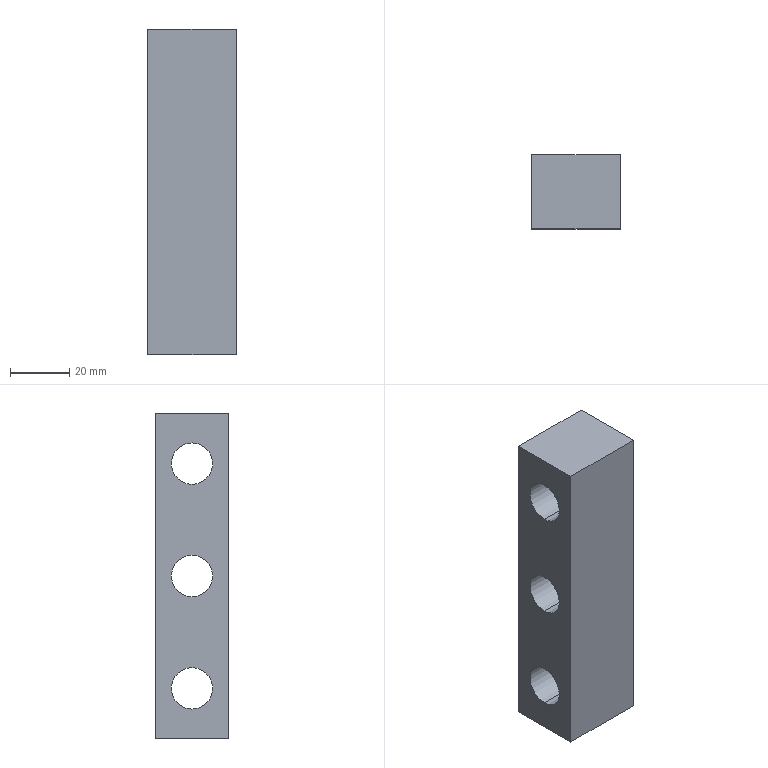Component | SolidWorks | CS021-A10-A005-3 | 1 solid | 44 faces | box 30 x 25 x 110 mm | volume 67025 mm3 | cylinder 22 | cone 16 | plane 6 | commonest cylinder face diameters 4.2 x16 14 x6 | material Q235
build123d program:
from build123d import *

# Parameters (mm, degrees)
SKETCH1_W             = 110
SKETCH1_H             = 25
BOSS_EXTRUDE1_DEPTH   = 15
SKETCH2_R             = 7
CUT_EXTRUDE1_DEPTH    = 64.885
M5_TAPPED_HOLE1_D     = 4.2
M5_TAPPED_HOLE1_DEPTH = 14
M5_TAPPED_HOLE1_TIP   = 1.262
M5_TAPPED_HOLE2_D     = 4.2
M5_TAPPED_HOLE2_DEPTH = 14.4
M5_TAPPED_HOLE2_TIP   = 1.262


with BuildPart() as part:
    # Sketch1 → Boss-Extrude1 (new, symmetric)
    with BuildSketch(Plane.XY):
        Rectangle(SKETCH1_W, SKETCH1_H)
    extrude(amount=BOSS_EXTRUDE1_DEPTH, both=True)

    # Sketch2 → Cut-Extrude1 (cut, through all)
    with BuildSketch(Plane.XY.offset(15)):
        with Locations((-38, 0)):
            Circle(SKETCH2_R)
        Circle(SKETCH2_R)
        with Locations(Location((38, 0, 0), (0, 0, 180))):
            Circle(SKETCH2_R)
    extrude(amount=-CUT_EXTRUDE1_DEPTH, mode=Mode.SUBTRACT)

    # M5 Tapped Hole1
    with Locations(Plane(origin=(0, 12.5, 0), x_dir=(1, 0, 0), z_dir=(0, 1, 0))):
        with Locations((15, 10), (15, -10), (-15, -10), (-15, 10)):
            Hole(M5_TAPPED_HOLE1_D / 2, depth=M5_TAPPED_HOLE1_DEPTH)
            with Locations((0, 0, -(M5_TAPPED_HOLE1_DEPTH + M5_TAPPED_HOLE1_TIP / 2))):  # 118° drill point
                Cone(0, M5_TAPPED_HOLE1_D / 2, M5_TAPPED_HOLE1_TIP, mode=Mode.SUBTRACT)

    # M5 Tapped Hole2
    with Locations(Plane(origin=(0, 12.5, 0), x_dir=(1, 0, 0), z_dir=(0, 1, 0))):
        with Locations((-25, 9), (25, 9), (25, -9), (-25, -9)):
            Hole(M5_TAPPED_HOLE2_D / 2, depth=M5_TAPPED_HOLE2_DEPTH)
            with Locations((0, 0, -(M5_TAPPED_HOLE2_DEPTH + M5_TAPPED_HOLE2_TIP / 2))):  # 118° drill point
                Cone(0, M5_TAPPED_HOLE2_D / 2, M5_TAPPED_HOLE2_TIP, mode=Mode.SUBTRACT)


solid = part.part

# Placed as in the assembly
solid = solid.moved(Location((152.449, 84.817, 0), (0, 90, 0)))